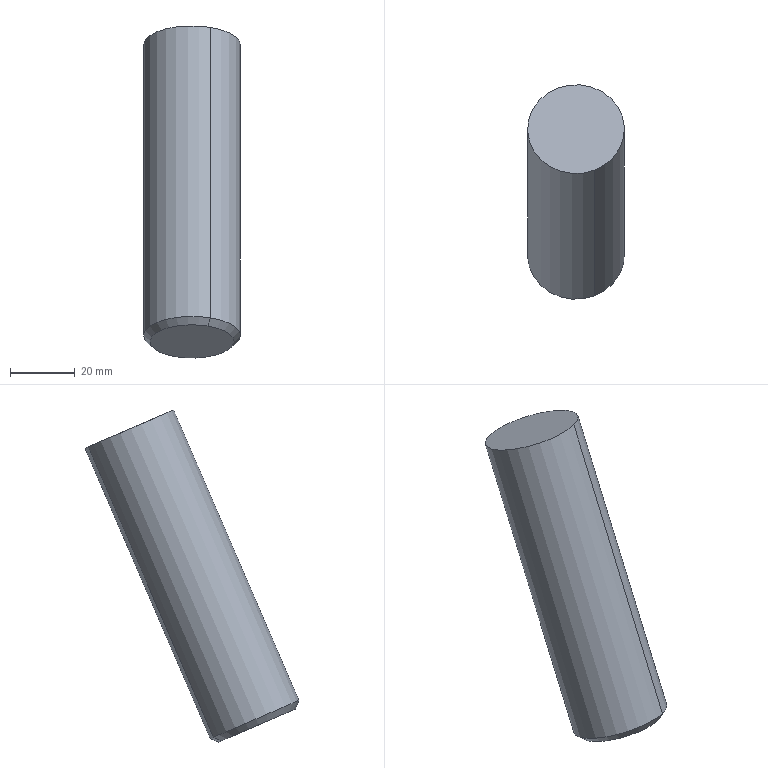Component | SolidWorks | Donja oslona ploca-10_Vijak donje oslone ploce-1 | 1 solid | 6 faces | box 30 x 66.35 x 102.91 mm | volume 70506 mm3 | cone 2 | cylinder 2 | plane 2 | commonest cylinder face diameters 30 x2
build123d program:
from build123d import *

# Parameters (mm, degrees)
SKETCH1_R           = 15
BOSS_EXTRUDE1_DEPTH = 100
CHAMFER1_SIZE       = 2


with BuildPart() as part:
    # Sketch1 → Boss-Extrude1 (new body)
    with BuildSketch(Plane(origin=(0, 0, 0), x_dir=(1, 0, 0), z_dir=(0, 1, 0))):
        with Locations(Location((0, 0, 0), (0, 0, 270))):
            Circle(SKETCH1_R)
    extrude(amount=BOSS_EXTRUDE1_DEPTH)

    # Chamfer1
    chamfer1_edges = [part.edges().sort_by_distance(p)[0] for p in [
        (0, 100, -15),
    ]]
    chamfer(chamfer1_edges, length=CHAMFER1_SIZE)


solid = part.part

# Placed as in the assembly
solid = solid.moved(Location((-677, -103.133, -239.215), (66.678, 0.3276, 180)))
STEP:
#1=COLOUR_RGB('',0.7922,0.8196,0.9333);
#2=FILL_AREA_STYLE_COLOUR('',#1);
#3=FILL_AREA_STYLE('',(#2));
#4=SURFACE_STYLE_FILL_AREA(#3);
#5=SURFACE_SIDE_STYLE('',(#4));
#6=SURFACE_STYLE_USAGE(.BOTH.,#5);
#7=PRESENTATION_STYLE_ASSIGNMENT((#6));
#8=CARTESIAN_POINT('',(-26.457,-6.053,-12.846));
#9=VERTEX_POINT('',#8);
#10=CARTESIAN_POINT('',(-26.85,-5.185,-13.22));
#11=VERTEX_POINT('',#10);
#12=CARTESIAN_POINT('',(-26.654,-5.619,-13.033));
#13=DIRECTION('',(-0.,-0.3959,-0.9183));
#14=DIRECTION('',(0.383,-0.8483,0.3657));
#15=AXIS2_PLACEMENT_3D('',#12,#13,#14);
#16=CIRCLE('',#15,0.5118);
#17=EDGE_CURVE('',#9,#11,#16,.T.);
#18=ORIENTED_EDGE('',*,*,#17,.F.);
#19=CARTESIAN_POINT('',(-26.427,-6.089,-12.745));
#20=VERTEX_POINT('',#19);
#21=CARTESIAN_POINT('',(-26.457,-6.053,-12.846));
#22=DIRECTION('',(0.2709,-0.3199,0.9079));
#23=VECTOR('',#22,39.37);
#24=LINE('',#21,#23);
#25=EDGE_CURVE('',#9,#20,#24,.T.);
#26=ORIENTED_EDGE('',*,*,#25,.T.);
#27=CARTESIAN_POINT('',(-26.88,-5.087,-13.177));
#28=VERTEX_POINT('',#27);
#29=CARTESIAN_POINT('',(-26.654,-5.588,-12.961));
#30=DIRECTION('',(0.,0.3959,0.9183));
#31=DIRECTION('',(0.383,-0.8483,0.3657));
#32=AXIS2_PLACEMENT_3D('',#29,#30,#31);
#33=CIRCLE('',#32,0.5906);
#34=EDGE_CURVE('',#28,#20,#33,.T.);
#35=ORIENTED_EDGE('',*,*,#34,.F.);
#36=CARTESIAN_POINT('',(-26.85,-5.185,-13.22));
#37=DIRECTION('',(-0.2709,0.8798,0.3907));
#38=VECTOR('',#37,39.37);
#39=LINE('',#36,#38);
#40=EDGE_CURVE('',#11,#28,#39,.T.);
#41=ORIENTED_EDGE('',*,*,#40,.F.);
#42=EDGE_LOOP('',(#18,#26,#35,#41));
#43=FACE_OUTER_BOUND('',#42,.T.);
#44=CARTESIAN_POINT('',(-26.654,-5.619,-13.033));
#45=DIRECTION('',(0.,0.3959,0.9183));
#46=DIRECTION('',(-0.383,0.8483,-0.3657));
#47=AXIS2_PLACEMENT_3D('',#44,#45,#46);
#48=CONICAL_SURFACE('',#47,0.5118,0.7854);
#49=ADVANCED_FACE('',(#43),#48,.T.);
#50=ORIENTED_EDGE('',*,*,#34,.T.);
#51=CARTESIAN_POINT('',(-26.427,-4.561,-9.202));
#52=VERTEX_POINT('',#51);
#53=CARTESIAN_POINT('',(-26.427,-6.12,-12.817));
#54=DIRECTION('',(0.,0.3959,0.9183));
#55=VECTOR('',#54,39.37);
#56=LINE('',#53,#55);
#57=EDGE_CURVE('',#20,#52,#56,.T.);
#58=ORIENTED_EDGE('',*,*,#57,.T.);
#59=CARTESIAN_POINT('',(-26.88,-3.559,-9.634));
#60=VERTEX_POINT('',#59);
#61=CARTESIAN_POINT('',(-26.654,-4.06,-9.418));
#62=DIRECTION('',(-0.,-0.3959,-0.9183));
#63=DIRECTION('',(0.383,-0.8483,0.3657));
#64=AXIS2_PLACEMENT_3D('',#61,#62,#63);
#65=CIRCLE('',#64,0.5906);
#66=EDGE_CURVE('',#52,#60,#65,.T.);
#67=ORIENTED_EDGE('',*,*,#66,.T.);
#68=CARTESIAN_POINT('',(-26.88,-5.118,-13.249));
#69=DIRECTION('',(0.,0.3959,0.9183));
#70=VECTOR('',#69,39.37);
#71=LINE('',#68,#70);
#72=EDGE_CURVE('',#28,#60,#71,.T.);
#73=ORIENTED_EDGE('',*,*,#72,.F.);
#74=EDGE_LOOP('',(#50,#58,#67,#73));
#75=FACE_OUTER_BOUND('',#74,.T.);
#76=CARTESIAN_POINT('',(-26.654,-5.619,-13.033));
#77=DIRECTION('',(0.,0.3959,0.9183));
#78=DIRECTION('',(-0.383,0.8483,-0.3657));
#79=AXIS2_PLACEMENT_3D('',#76,#77,#78);
#80=CYLINDRICAL_SURFACE('',#79,0.5906);
#81=ADVANCED_FACE('',(#75),#80,.T.);
#82=ORIENTED_EDGE('',*,*,#57,.F.);
#83=CARTESIAN_POINT('',(-26.654,-5.588,-12.961));
#84=DIRECTION('',(0.,0.3959,0.9183));
#85=DIRECTION('',(0.383,-0.8483,0.3657));
#86=AXIS2_PLACEMENT_3D('',#83,#84,#85);
#87=CIRCLE('',#86,0.5906);
#88=EDGE_CURVE('',#20,#28,#87,.T.);
#89=ORIENTED_EDGE('',*,*,#88,.T.);
#90=ORIENTED_EDGE('',*,*,#72,.T.);
#91=CARTESIAN_POINT('',(-26.654,-4.06,-9.418));
#92=DIRECTION('',(-0.,-0.3959,-0.9183));
#93=DIRECTION('',(0.383,-0.8483,0.3657));
#94=AXIS2_PLACEMENT_3D('',#91,#92,#93);
#95=CIRCLE('',#94,0.5906);
#96=EDGE_CURVE('',#60,#52,#95,.T.);
#97=ORIENTED_EDGE('',*,*,#96,.T.);
#98=EDGE_LOOP('',(#82,#89,#90,#97));
#99=FACE_OUTER_BOUND('',#98,.T.);
#100=CARTESIAN_POINT('',(-26.654,-5.619,-13.033));
#101=DIRECTION('',(0.,0.3959,0.9183));
#102=DIRECTION('',(-0.383,0.8483,-0.3657));
#103=AXIS2_PLACEMENT_3D('',#100,#101,#102);
#104=CYLINDRICAL_SURFACE('',#103,0.5906);
#105=ADVANCED_FACE('',(#99),#104,.T.);
#106=CARTESIAN_POINT('',(-26.654,-5.619,-13.033));
#107=DIRECTION('',(-0.,-0.3959,-0.9183));
#108=DIRECTION('',(0.383,-0.8483,0.3657));
#109=AXIS2_PLACEMENT_3D('',#106,#107,#108);
#110=CIRCLE('',#109,0.5118);
#111=EDGE_CURVE('',#11,#9,#110,.T.);
#112=ORIENTED_EDGE('',*,*,#111,.T.);
#113=ORIENTED_EDGE('',*,*,#17,.T.);
#114=EDGE_LOOP('',(#112,#113));
#115=FACE_OUTER_BOUND('',#114,.T.);
#116=CARTESIAN_POINT('',(-26.654,-5.619,-13.033));
#117=DIRECTION('',(-0.,-0.3959,-0.9183));
#118=DIRECTION('',(0.383,-0.8483,0.3657));
#119=AXIS2_PLACEMENT_3D('',#116,#117,#118);
#120=PLANE('',#119);
#121=ADVANCED_FACE('',(#115),#120,.T.);
#122=ORIENTED_EDGE('',*,*,#96,.F.);
#123=ORIENTED_EDGE('',*,*,#66,.F.);
#124=EDGE_LOOP('',(#122,#123));
#125=FACE_OUTER_BOUND('',#124,.T.);
#126=CARTESIAN_POINT('',(-26.654,-4.06,-9.418));
#127=DIRECTION('',(-0.,-0.3959,-0.9183));
#128=DIRECTION('',(0.383,-0.8483,0.3657));
#129=AXIS2_PLACEMENT_3D('',#126,#127,#128);
#130=PLANE('',#129);
#131=ADVANCED_FACE('',(#125),#130,.F.);
#132=ORIENTED_EDGE('',*,*,#25,.F.);
#133=ORIENTED_EDGE('',*,*,#111,.F.);
#134=ORIENTED_EDGE('',*,*,#40,.T.);
#135=ORIENTED_EDGE('',*,*,#88,.F.);
#136=EDGE_LOOP('',(#132,#133,#134,#135));
#137=FACE_OUTER_BOUND('',#136,.T.);
#138=CARTESIAN_POINT('',(-26.654,-5.619,-13.033));
#139=DIRECTION('',(0.,0.3959,0.9183));
#140=DIRECTION('',(-0.383,0.8483,-0.3657));
#141=AXIS2_PLACEMENT_3D('',#138,#139,#140);
#142=CONICAL_SURFACE('',#141,0.5118,0.7854);
#143=ADVANCED_FACE('',(#137),#142,.T.);
#144=CLOSED_SHELL('',(#49,#81,#105,#121,#131,#143));
#145=MANIFOLD_SOLID_BREP('',#144);
#146=STYLED_ITEM('',(#7),#145);
#147=(LENGTH_UNIT()NAMED_UNIT(*)SI_UNIT($,.METRE.));
#148=LENGTH_MEASURE_WITH_UNIT(LENGTH_MEASURE(0.0254),#147);
#149=DIMENSIONAL_EXPONENTS(1.,0.,0.,0.,0.,0.,0.);
#150=(CONVERSION_BASED_UNIT('',#148)LENGTH_UNIT()NAMED_UNIT(#149));
#151=UNCERTAINTY_MEASURE_WITH_UNIT(LENGTH_MEASURE(0.00001),#150,'','');
#152=(NAMED_UNIT(*)PLANE_ANGLE_UNIT()SI_UNIT($,.RADIAN.));
#153=(NAMED_UNIT(*)SI_UNIT($,.STERADIAN.)SOLID_ANGLE_UNIT());
#154=(GEOMETRIC_REPRESENTATION_CONTEXT(3)GLOBAL_UNCERTAINTY_ASSIGNED_CONTEXT((#151))GLOBAL_UNIT_ASSIGNED_CONTEXT((#150,#152,#153))REPRESENTATION_CONTEXT('',''));
#155=MECHANICAL_DESIGN_GEOMETRIC_PRESENTATION_REPRESENTATION('',(#146),#154);
#156=PRESENTATION_LAYER_ASSIGNMENT('','',(#146));
#157=CARTESIAN_POINT('',(0.,0.,0.));
#158=DIRECTION('',(0.,0.,1.));
#159=DIRECTION('',(1.,0.,0.));
#160=AXIS2_PLACEMENT_3D('',#157,#158,#159);
#161=(LENGTH_UNIT()NAMED_UNIT(*)SI_UNIT($,.METRE.));
#162=LENGTH_MEASURE_WITH_UNIT(LENGTH_MEASURE(0.0254),#161);
#163=DIMENSIONAL_EXPONENTS(1.,0.,0.,0.,0.,0.,0.);
#164=(CONVERSION_BASED_UNIT('',#162)LENGTH_UNIT()NAMED_UNIT(#163));
#165=UNCERTAINTY_MEASURE_WITH_UNIT(LENGTH_MEASURE(0.00001),#164,'','');
#166=(NAMED_UNIT(*)PLANE_ANGLE_UNIT()SI_UNIT($,.RADIAN.));
#167=(NAMED_UNIT(*)SI_UNIT($,.STERADIAN.)SOLID_ANGLE_UNIT());
#168=(GEOMETRIC_REPRESENTATION_CONTEXT(3)GLOBAL_UNCERTAINTY_ASSIGNED_CONTEXT((#165))GLOBAL_UNIT_ASSIGNED_CONTEXT((#164,#166,#167))REPRESENTATION_CONTEXT('',''));
#169=ADVANCED_BREP_SHAPE_REPRESENTATION('',(#145,#160),#168);